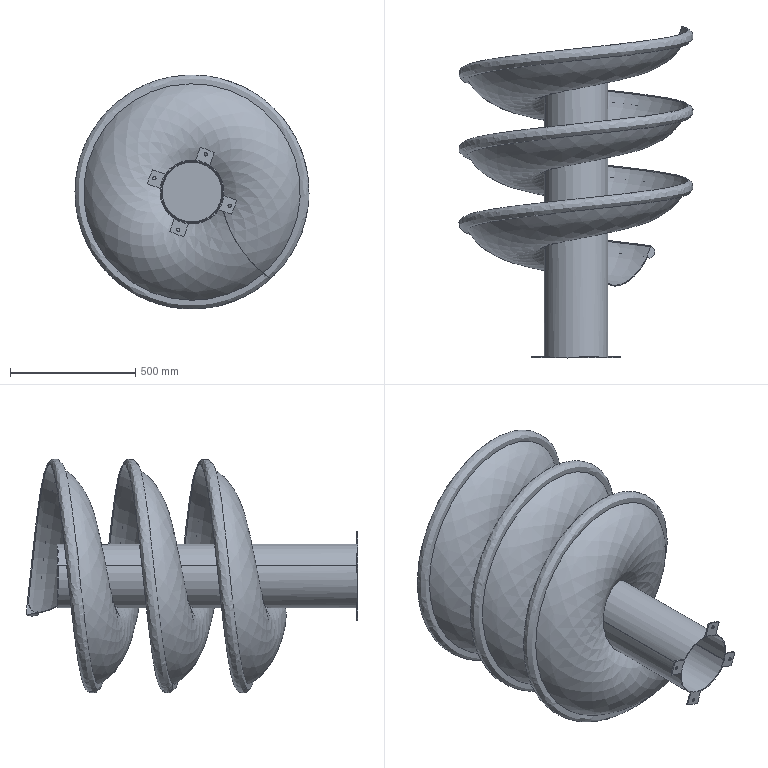Component | SolidWorks | 02-01RollingTrack-1 | 1 solid | 56 faces | volume 18167220 mm3 | cylinder 27 | plane 16 | spline 13 | commonest cylinder face diameters 13.5 x8 249 x7 255 x6 360 x5 948.149 x1